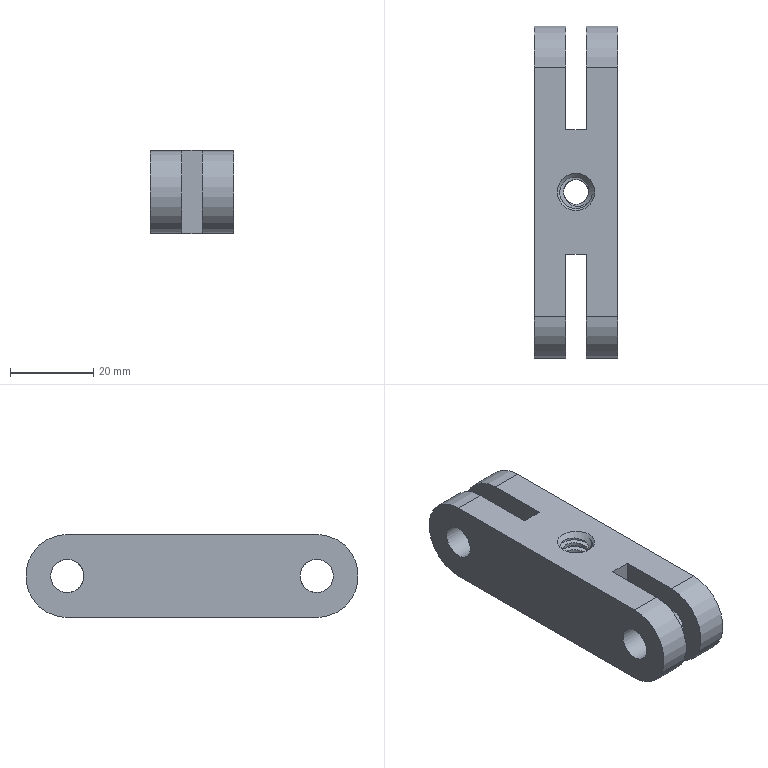Component | NX | PUSHPLATE | 1 solid | 24 faces | volume 23379 mm3 | cylinder 10 | plane 10 | cone 2 | spline 2 | commonest cylinder face diameters 8 x5 20 x4 6 x1